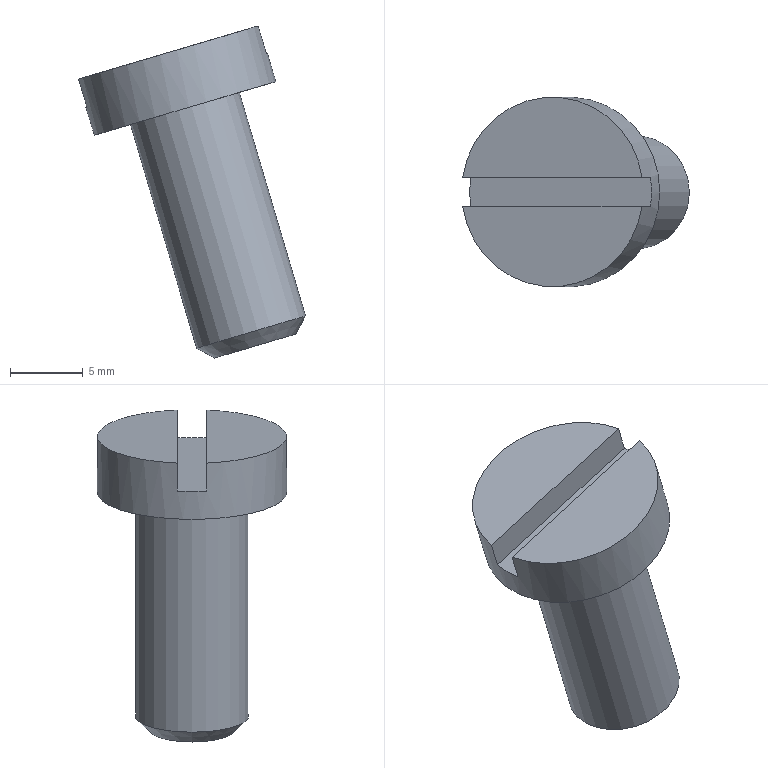Component | NX | SCREW_M8 | 1 solid | 10 faces | box 15.56 x 13 x 22.78 mm | volume 1277 mm3 | plane 7 | cylinder 2 | cone 1 | commonest cylinder face diameters 13 x1 7.785 x1
STEP:
#1=CARTESIAN_POINT('',(0.,0.,0.));
#2=DIRECTION('',(0.,0.,1.));
#3=DIRECTION('',(1.,0.,0.));
#4=AXIS2_PLACEMENT_3D('',#1,#2,#3);
#5=CARTESIAN_POINT('',(95.853,-1.,167.137));
#6=VERTEX_POINT('',#5);
#7=CARTESIAN_POINT('',(108.171,-1.,170.779));
#8=VERTEX_POINT('',#7);
#9=CARTESIAN_POINT('',(102.012,0.,168.958));
#10=DIRECTION('',(-0.2835,0.,0.959));
#11=DIRECTION('',(0.959,0.,0.2835));
#12=AXIS2_PLACEMENT_3D('',#9,#10,#11);
#13=CIRCLE('',#12,6.5);
#14=CARTESIAN_POINT('',(102.012,0.,168.958));
#15=DIRECTION('',(-0.2835,0.,0.959));
#16=DIRECTION('',(0.959,0.,0.2835));
#17=AXIS2_PLACEMENT_3D('',#14,#15,#16);
#18=PLANE('',#17);
#19=CARTESIAN_POINT('',(0.,0.));
#20=DIRECTION('',(1.,0.));
#21=AXIS2_PLACEMENT_2D('',#19,#20);
#22=CIRCLE('',#21,6.5);
#23=(GEOMETRIC_REPRESENTATION_CONTEXT(2)PARAMETRIC_REPRESENTATION_CONTEXT()REPRESENTATION_CONTEXT('',''));
#24=DEFINITIONAL_REPRESENTATION('',(#22),#23);
#25=PCURVE('',#18,#24);
#26=CARTESIAN_POINT('',(103.146,0.,165.122));
#27=DIRECTION('',(-0.2835,0.,0.959));
#28=DIRECTION('',(0.959,0.,0.2835));
#29=AXIS2_PLACEMENT_3D('',#26,#27,#28);
#30=CYLINDRICAL_SURFACE('',#29,6.5);
#31=CARTESIAN_POINT('',(0.,4.));
#32=DIRECTION('',(1.,0.));
#33=VECTOR('',#32,1.);
#34=LINE('',#31,#33);
#35=(GEOMETRIC_REPRESENTATION_CONTEXT(2)PARAMETRIC_REPRESENTATION_CONTEXT()REPRESENTATION_CONTEXT('',''));
#36=DEFINITIONAL_REPRESENTATION('',(#34),#35);
#37=PCURVE('',#30,#36);
#38=SURFACE_CURVE('',#13,(#25,#37),.PCURVE_S1.);
#39=EDGE_CURVE('',#6,#8,#38,.T.);
#40=ORIENTED_EDGE('',*,*,#39,.T.);
#41=CARTESIAN_POINT('',(111.193,-1.,171.672));
#42=DIRECTION('',(-0.959,0.,-0.2835));
#43=VECTOR('',#42,1.);
#44=LINE('',#41,#43);
#45=CARTESIAN_POINT('',(9.574,-1.));
#46=DIRECTION('',(-1.,0.));
#47=VECTOR('',#46,1.);
#48=LINE('',#45,#47);
#49=(GEOMETRIC_REPRESENTATION_CONTEXT(2)PARAMETRIC_REPRESENTATION_CONTEXT()REPRESENTATION_CONTEXT('',''));
#50=DEFINITIONAL_REPRESENTATION('',(#48),#49);
#51=PCURVE('',#18,#50);
#52=CARTESIAN_POINT('',(111.76,-1.,169.754));
#53=DIRECTION('',(0.,1.,0.));
#54=DIRECTION('',(-0.2835,0.,0.959));
#55=AXIS2_PLACEMENT_3D('',#52,#53,#54);
#56=PLANE('',#55);
#57=CARTESIAN_POINT('',(2.,0.));
#58=DIRECTION('',(0.,-1.));
#59=VECTOR('',#58,1.);
#60=LINE('',#57,#59);
#61=(GEOMETRIC_REPRESENTATION_CONTEXT(2)PARAMETRIC_REPRESENTATION_CONTEXT()REPRESENTATION_CONTEXT('',''));
#62=DEFINITIONAL_REPRESENTATION('',(#60),#61);
#63=PCURVE('',#56,#62);
#64=SURFACE_CURVE('',#44,(#51,#63),.PCURVE_S1.);
#65=EDGE_CURVE('',#8,#6,#64,.T.);
#66=ORIENTED_EDGE('',*,*,#65,.T.);
#67=EDGE_LOOP('',(#40,#66));
#68=FACE_BOUND('',#67,.T.);
#69=ADVANCED_FACE('',(#68),#18,.T.);
#70=CARTESIAN_POINT('',(108.171,1.,170.779));
#71=VERTEX_POINT('',#70);
#72=CARTESIAN_POINT('',(95.853,1.,167.137));
#73=VERTEX_POINT('',#72);
#74=CARTESIAN_POINT('',(102.012,0.,168.958));
#75=DIRECTION('',(-0.2835,0.,0.959));
#76=DIRECTION('',(0.959,0.,0.2835));
#77=AXIS2_PLACEMENT_3D('',#74,#75,#76);
#78=CIRCLE('',#77,6.5);
#79=CARTESIAN_POINT('',(102.012,0.,168.958));
#80=DIRECTION('',(-0.2835,0.,0.959));
#81=DIRECTION('',(0.959,0.,0.2835));
#82=AXIS2_PLACEMENT_3D('',#79,#80,#81);
#83=PLANE('',#82);
#84=CARTESIAN_POINT('',(0.,0.));
#85=DIRECTION('',(1.,0.));
#86=AXIS2_PLACEMENT_2D('',#84,#85);
#87=CIRCLE('',#86,6.5);
#88=(GEOMETRIC_REPRESENTATION_CONTEXT(2)PARAMETRIC_REPRESENTATION_CONTEXT()REPRESENTATION_CONTEXT('',''));
#89=DEFINITIONAL_REPRESENTATION('',(#87),#88);
#90=PCURVE('',#83,#89);
#91=CARTESIAN_POINT('',(-0.,4.));
#92=DIRECTION('',(1.,-0.));
#93=VECTOR('',#92,1.);
#94=LINE('',#91,#93);
#95=(GEOMETRIC_REPRESENTATION_CONTEXT(2)PARAMETRIC_REPRESENTATION_CONTEXT()REPRESENTATION_CONTEXT('',''));
#96=DEFINITIONAL_REPRESENTATION('',(#94),#95);
#97=PCURVE('',#30,#96);
#98=SURFACE_CURVE('',#78,(#90,#97),.PCURVE_S1.);
#99=EDGE_CURVE('',#71,#73,#98,.T.);
#100=ORIENTED_EDGE('',*,*,#99,.T.);
#101=CARTESIAN_POINT('',(92.831,1.,166.243));
#102=DIRECTION('',(0.959,0.,0.2835));
#103=VECTOR('',#102,1.);
#104=LINE('',#101,#103);
#105=CARTESIAN_POINT('',(-9.574,1.));
#106=DIRECTION('',(1.,0.));
#107=VECTOR('',#106,1.);
#108=LINE('',#105,#107);
#109=(GEOMETRIC_REPRESENTATION_CONTEXT(2)PARAMETRIC_REPRESENTATION_CONTEXT()REPRESENTATION_CONTEXT('',''));
#110=DEFINITIONAL_REPRESENTATION('',(#108),#109);
#111=PCURVE('',#83,#110);
#112=CARTESIAN_POINT('',(93.398,1.,164.325));
#113=DIRECTION('',(0.,-1.,0.));
#114=DIRECTION('',(0.2835,0.,-0.959));
#115=AXIS2_PLACEMENT_3D('',#112,#113,#114);
#116=PLANE('',#115);
#117=CARTESIAN_POINT('',(-2.,-0.));
#118=DIRECTION('',(0.,1.));
#119=VECTOR('',#118,1.);
#120=LINE('',#117,#119);
#121=(GEOMETRIC_REPRESENTATION_CONTEXT(2)PARAMETRIC_REPRESENTATION_CONTEXT()REPRESENTATION_CONTEXT('',''));
#122=DEFINITIONAL_REPRESENTATION('',(#120),#121);
#123=PCURVE('',#116,#122);
#124=SURFACE_CURVE('',#104,(#111,#123),.PCURVE_S1.);
#125=EDGE_CURVE('',#73,#71,#124,.T.);
#126=ORIENTED_EDGE('',*,*,#125,.T.);
#127=EDGE_LOOP('',(#100,#126));
#128=FACE_BOUND('',#127,.T.);
#129=ADVANCED_FACE('',(#128),#83,.T.);
#130=CARTESIAN_POINT('',(109.38,0.,166.965));
#131=VERTEX_POINT('',#130);
#132=CARTESIAN_POINT('',(103.146,0.,165.122));
#133=DIRECTION('',(-0.2835,0.,0.959));
#134=DIRECTION('',(0.959,0.,0.2835));
#135=AXIS2_PLACEMENT_3D('',#132,#133,#134);
#136=CIRCLE('',#135,6.5);
#137=CARTESIAN_POINT('',(0.,0.));
#138=DIRECTION('',(1.,0.));
#139=VECTOR('',#138,1.);
#140=LINE('',#137,#139);
#141=(GEOMETRIC_REPRESENTATION_CONTEXT(2)PARAMETRIC_REPRESENTATION_CONTEXT()REPRESENTATION_CONTEXT('',''));
#142=DEFINITIONAL_REPRESENTATION('',(#140),#141);
#143=PCURVE('',#30,#142);
#144=CARTESIAN_POINT('',(103.146,0.,165.122));
#145=DIRECTION('',(0.2835,0.,-0.959));
#146=DIRECTION('',(-0.959,0.,-0.2835));
#147=AXIS2_PLACEMENT_3D('',#144,#145,#146);
#148=PLANE('',#147);
#149=CARTESIAN_POINT('',(-6.5,0.));
#150=CARTESIAN_POINT('',(-6.5,11.258));
#151=CARTESIAN_POINT('',(3.25,5.629));
#152=CARTESIAN_POINT('',(13.,0.));
#153=CARTESIAN_POINT('',(3.25,-5.629));
#154=CARTESIAN_POINT('',(-6.5,-11.258));
#155=CARTESIAN_POINT('',(-6.5,0.));
#156=(BOUNDED_CURVE()B_SPLINE_CURVE(2,(#149,#150,#151,#152,#153,#154,#155),.UNSPECIFIED.,.T.,.F.)B_SPLINE_CURVE_WITH_KNOTS((1,2,2,2,2,1),(-2.094,0.,2.094,4.189,6.283,8.378),.UNSPECIFIED.)CURVE()GEOMETRIC_REPRESENTATION_ITEM()RATIONAL_B_SPLINE_CURVE((1.,0.5,1.,0.5,1.,0.5,1.))REPRESENTATION_ITEM(''));
#157=(GEOMETRIC_REPRESENTATION_CONTEXT(2)PARAMETRIC_REPRESENTATION_CONTEXT()REPRESENTATION_CONTEXT('',''));
#158=DEFINITIONAL_REPRESENTATION('',(#156),#157);
#159=PCURVE('',#148,#158);
#160=SURFACE_CURVE('',#136,(#143,#159),.PCURVE_S1.);
#161=EDGE_CURVE('',#131,#131,#160,.T.);
#162=ORIENTED_EDGE('',*,*,#161,.T.);
#163=CARTESIAN_POINT('',(108.812,0.,168.883));
#164=VERTEX_POINT('',#163);
#165=CARTESIAN_POINT('',(109.38,0.,166.965));
#166=CARTESIAN_POINT('',(108.812,0.,168.883));
#167=B_SPLINE_CURVE_WITH_KNOTS('',1,(#165,#166),.UNSPECIFIED.,.F.,.F.,(2,2),(0.,2.),.PIECEWISE_BEZIER_KNOTS.);
#168=CARTESIAN_POINT('',(6.283,0.));
#169=DIRECTION('',(0.,1.));
#170=VECTOR('',#169,1.);
#171=LINE('',#168,#170);
#172=(GEOMETRIC_REPRESENTATION_CONTEXT(2)PARAMETRIC_REPRESENTATION_CONTEXT()REPRESENTATION_CONTEXT('',''));
#173=DEFINITIONAL_REPRESENTATION('',(#171),#172);
#174=PCURVE('',#30,#173);
#175=CARTESIAN_POINT('',(0.,0.));
#176=DIRECTION('',(0.,1.));
#177=VECTOR('',#176,1.);
#178=LINE('',#175,#177);
#179=(GEOMETRIC_REPRESENTATION_CONTEXT(2)PARAMETRIC_REPRESENTATION_CONTEXT()REPRESENTATION_CONTEXT('',''));
#180=DEFINITIONAL_REPRESENTATION('',(#178),#179);
#181=PCURVE('',#30,#180);
#182=SEAM_CURVE('',#167,(#174,#181),.PCURVE_S1.);
#183=EDGE_CURVE('',#131,#164,#182,.T.);
#184=ORIENTED_EDGE('',*,*,#183,.T.);
#185=CARTESIAN_POINT('',(108.738,-1.,168.861));
#186=VERTEX_POINT('',#185);
#187=CARTESIAN_POINT('',(102.579,0.,167.04));
#188=DIRECTION('',(-0.2835,0.,0.959));
#189=DIRECTION('',(-0.959,0.,-0.2835));
#190=AXIS2_PLACEMENT_3D('',#187,#188,#189);
#191=CIRCLE('',#190,6.5);
#192=CARTESIAN_POINT('',(3.142,2.));
#193=DIRECTION('',(1.,0.));
#194=VECTOR('',#193,1.);
#195=LINE('',#192,#194);
#196=(GEOMETRIC_REPRESENTATION_CONTEXT(2)PARAMETRIC_REPRESENTATION_CONTEXT()REPRESENTATION_CONTEXT('',''));
#197=DEFINITIONAL_REPRESENTATION('',(#195),#196);
#198=PCURVE('',#30,#197);
#199=CARTESIAN_POINT('',(102.579,0.,167.04));
#200=DIRECTION('',(0.2835,0.,-0.959));
#201=DIRECTION('',(-0.959,0.,-0.2835));
#202=AXIS2_PLACEMENT_3D('',#199,#200,#201);
#203=PLANE('',#202);
#204=CARTESIAN_POINT('',(6.5,0.));
#205=CARTESIAN_POINT('',(6.5,-11.258));
#206=CARTESIAN_POINT('',(-3.25,-5.629));
#207=CARTESIAN_POINT('',(-13.,-0.));
#208=CARTESIAN_POINT('',(-3.25,5.629));
#209=CARTESIAN_POINT('',(6.5,11.258));
#210=CARTESIAN_POINT('',(6.5,0.));
#211=(BOUNDED_CURVE()B_SPLINE_CURVE(2,(#204,#205,#206,#207,#208,#209,#210),.UNSPECIFIED.,.T.,.F.)B_SPLINE_CURVE_WITH_KNOTS((1,2,2,2,2,1),(-2.094,0.,2.094,4.189,6.283,8.378),.UNSPECIFIED.)CURVE()GEOMETRIC_REPRESENTATION_ITEM()RATIONAL_B_SPLINE_CURVE((1.,0.5,1.,0.5,1.,0.5,1.))REPRESENTATION_ITEM(''));
#212=(GEOMETRIC_REPRESENTATION_CONTEXT(2)PARAMETRIC_REPRESENTATION_CONTEXT()REPRESENTATION_CONTEXT('',''));
#213=DEFINITIONAL_REPRESENTATION('',(#211),#212);
#214=PCURVE('',#203,#213);
#215=SURFACE_CURVE('',#191,(#198,#214),.PCURVE_S1.);
#216=EDGE_CURVE('',#186,#164,#215,.T.);
#217=ORIENTED_EDGE('',*,*,#216,.F.);
#218=CARTESIAN_POINT('',(109.305,-1.,166.943));
#219=DIRECTION('',(-0.2835,0.,0.959));
#220=VECTOR('',#219,1.);
#221=LINE('',#218,#220);
#222=CARTESIAN_POINT('',(6.129,-0.));
#223=DIRECTION('',(0.,1.));
#224=VECTOR('',#223,1.);
#225=LINE('',#222,#224);
#226=(GEOMETRIC_REPRESENTATION_CONTEXT(2)PARAMETRIC_REPRESENTATION_CONTEXT()REPRESENTATION_CONTEXT('',''));
#227=DEFINITIONAL_REPRESENTATION('',(#225),#226);
#228=PCURVE('',#30,#227);
#229=CARTESIAN_POINT('',(-2.,-3.151));
#230=DIRECTION('',(1.,0.));
#231=VECTOR('',#230,1.);
#232=LINE('',#229,#231);
#233=(GEOMETRIC_REPRESENTATION_CONTEXT(2)PARAMETRIC_REPRESENTATION_CONTEXT()REPRESENTATION_CONTEXT('',''));
#234=DEFINITIONAL_REPRESENTATION('',(#232),#233);
#235=PCURVE('',#56,#234);
#236=SURFACE_CURVE('',#221,(#228,#235),.PCURVE_S1.);
#237=EDGE_CURVE('',#186,#8,#236,.T.);
#238=ORIENTED_EDGE('',*,*,#237,.T.);
#239=ORIENTED_EDGE('',*,*,#39,.F.);
#240=CARTESIAN_POINT('',(96.42,-1.,165.219));
#241=VERTEX_POINT('',#240);
#242=CARTESIAN_POINT('',(96.987,-1.,163.301));
#243=DIRECTION('',(0.2835,0.,-0.959));
#244=VECTOR('',#243,1.);
#245=LINE('',#242,#244);
#246=CARTESIAN_POINT('',(3.296,-0.));
#247=DIRECTION('',(0.,-1.));
#248=VECTOR('',#247,1.);
#249=LINE('',#246,#248);
#250=(GEOMETRIC_REPRESENTATION_CONTEXT(2)PARAMETRIC_REPRESENTATION_CONTEXT()REPRESENTATION_CONTEXT('',''));
#251=DEFINITIONAL_REPRESENTATION('',(#249),#250);
#252=PCURVE('',#30,#251);
#253=CARTESIAN_POINT('',(-2.,-15.996));
#254=DIRECTION('',(-1.,0.));
#255=VECTOR('',#254,1.);
#256=LINE('',#253,#255);
#257=(GEOMETRIC_REPRESENTATION_CONTEXT(2)PARAMETRIC_REPRESENTATION_CONTEXT()REPRESENTATION_CONTEXT('',''));
#258=DEFINITIONAL_REPRESENTATION('',(#256),#257);
#259=PCURVE('',#56,#258);
#260=SURFACE_CURVE('',#245,(#252,#259),.PCURVE_S1.);
#261=EDGE_CURVE('',#6,#241,#260,.T.);
#262=ORIENTED_EDGE('',*,*,#261,.T.);
#263=CARTESIAN_POINT('',(96.42,1.,165.219));
#264=VERTEX_POINT('',#263);
#265=CARTESIAN_POINT('',(102.579,0.,167.04));
#266=DIRECTION('',(-0.2835,0.,0.959));
#267=DIRECTION('',(-0.959,0.,-0.2835));
#268=AXIS2_PLACEMENT_3D('',#265,#266,#267);
#269=CIRCLE('',#268,6.5);
#270=CARTESIAN_POINT('',(-3.142,2.));
#271=DIRECTION('',(1.,0.));
#272=VECTOR('',#271,1.);
#273=LINE('',#270,#272);
#274=(GEOMETRIC_REPRESENTATION_CONTEXT(2)PARAMETRIC_REPRESENTATION_CONTEXT()REPRESENTATION_CONTEXT('',''));
#275=DEFINITIONAL_REPRESENTATION('',(#273),#274);
#276=PCURVE('',#30,#275);
#277=CARTESIAN_POINT('',(6.5,0.));
#278=CARTESIAN_POINT('',(6.5,-11.258));
#279=CARTESIAN_POINT('',(-3.25,-5.629));
#280=CARTESIAN_POINT('',(-13.,-0.));
#281=CARTESIAN_POINT('',(-3.25,5.629));
#282=CARTESIAN_POINT('',(6.5,11.258));
#283=CARTESIAN_POINT('',(6.5,0.));
#284=(BOUNDED_CURVE()B_SPLINE_CURVE(2,(#277,#278,#279,#280,#281,#282,#283),.UNSPECIFIED.,.T.,.F.)B_SPLINE_CURVE_WITH_KNOTS((1,2,2,2,2,1),(-2.094,0.,2.094,4.189,6.283,8.378),.UNSPECIFIED.)CURVE()GEOMETRIC_REPRESENTATION_ITEM()RATIONAL_B_SPLINE_CURVE((1.,0.5,1.,0.5,1.,0.5,1.))REPRESENTATION_ITEM(''));
#285=(GEOMETRIC_REPRESENTATION_CONTEXT(2)PARAMETRIC_REPRESENTATION_CONTEXT()REPRESENTATION_CONTEXT('',''));
#286=DEFINITIONAL_REPRESENTATION('',(#284),#285);
#287=PCURVE('',#203,#286);
#288=SURFACE_CURVE('',#269,(#276,#287),.PCURVE_S1.);
#289=EDGE_CURVE('',#264,#241,#288,.T.);
#290=ORIENTED_EDGE('',*,*,#289,.F.);
#291=CARTESIAN_POINT('',(96.987,1.,163.301));
#292=DIRECTION('',(-0.2835,0.,0.959));
#293=VECTOR('',#292,1.);
#294=LINE('',#291,#293);
#295=CARTESIAN_POINT('',(2.987,-0.));
#296=DIRECTION('',(0.,1.));
#297=VECTOR('',#296,1.);
#298=LINE('',#295,#297);
#299=(GEOMETRIC_REPRESENTATION_CONTEXT(2)PARAMETRIC_REPRESENTATION_CONTEXT()REPRESENTATION_CONTEXT('',''));
#300=DEFINITIONAL_REPRESENTATION('',(#298),#299);
#301=PCURVE('',#30,#300);
#302=CARTESIAN_POINT('',(2.,3.151));
#303=DIRECTION('',(-1.,0.));
#304=VECTOR('',#303,1.);
#305=LINE('',#302,#304);
#306=(GEOMETRIC_REPRESENTATION_CONTEXT(2)PARAMETRIC_REPRESENTATION_CONTEXT()REPRESENTATION_CONTEXT('',''));
#307=DEFINITIONAL_REPRESENTATION('',(#305),#306);
#308=PCURVE('',#116,#307);
#309=SURFACE_CURVE('',#294,(#301,#308),.PCURVE_S1.);
#310=EDGE_CURVE('',#264,#73,#309,.T.);
#311=ORIENTED_EDGE('',*,*,#310,.T.);
#312=ORIENTED_EDGE('',*,*,#99,.F.);
#313=CARTESIAN_POINT('',(108.738,1.,168.861));
#314=VERTEX_POINT('',#313);
#315=CARTESIAN_POINT('',(109.305,1.,166.943));
#316=DIRECTION('',(0.2835,0.,-0.959));
#317=VECTOR('',#316,1.);
#318=LINE('',#315,#317);
#319=CARTESIAN_POINT('',(0.1545,-0.));
#320=DIRECTION('',(0.,-1.));
#321=VECTOR('',#320,1.);
#322=LINE('',#319,#321);
#323=(GEOMETRIC_REPRESENTATION_CONTEXT(2)PARAMETRIC_REPRESENTATION_CONTEXT()REPRESENTATION_CONTEXT('',''));
#324=DEFINITIONAL_REPRESENTATION('',(#322),#323);
#325=PCURVE('',#30,#324);
#326=CARTESIAN_POINT('',(2.,15.996));
#327=DIRECTION('',(1.,0.));
#328=VECTOR('',#327,1.);
#329=LINE('',#326,#328);
#330=(GEOMETRIC_REPRESENTATION_CONTEXT(2)PARAMETRIC_REPRESENTATION_CONTEXT()REPRESENTATION_CONTEXT('',''));
#331=DEFINITIONAL_REPRESENTATION('',(#329),#330);
#332=PCURVE('',#116,#331);
#333=SURFACE_CURVE('',#318,(#325,#332),.PCURVE_S1.);
#334=EDGE_CURVE('',#71,#314,#333,.T.);
#335=ORIENTED_EDGE('',*,*,#334,.T.);
#336=CARTESIAN_POINT('',(102.579,0.,167.04));
#337=DIRECTION('',(-0.2835,0.,0.959));
#338=DIRECTION('',(-0.959,0.,-0.2835));
#339=AXIS2_PLACEMENT_3D('',#336,#337,#338);
#340=CIRCLE('',#339,6.5);
#341=CARTESIAN_POINT('',(-3.142,2.));
#342=DIRECTION('',(1.,0.));
#343=VECTOR('',#342,1.);
#344=LINE('',#341,#343);
#345=(GEOMETRIC_REPRESENTATION_CONTEXT(2)PARAMETRIC_REPRESENTATION_CONTEXT()REPRESENTATION_CONTEXT('',''));
#346=DEFINITIONAL_REPRESENTATION('',(#344),#345);
#347=PCURVE('',#30,#346);
#348=CARTESIAN_POINT('',(6.5,0.));
#349=CARTESIAN_POINT('',(6.5,-11.258));
#350=CARTESIAN_POINT('',(-3.25,-5.629));
#351=CARTESIAN_POINT('',(-13.,-0.));
#352=CARTESIAN_POINT('',(-3.25,5.629));
#353=CARTESIAN_POINT('',(6.5,11.258));
#354=CARTESIAN_POINT('',(6.5,0.));
#355=(BOUNDED_CURVE()B_SPLINE_CURVE(2,(#348,#349,#350,#351,#352,#353,#354),.UNSPECIFIED.,.T.,.F.)B_SPLINE_CURVE_WITH_KNOTS((1,2,2,2,2,1),(-2.094,0.,2.094,4.189,6.283,8.378),.UNSPECIFIED.)CURVE()GEOMETRIC_REPRESENTATION_ITEM()RATIONAL_B_SPLINE_CURVE((1.,0.5,1.,0.5,1.,0.5,1.))REPRESENTATION_ITEM(''));
#356=(GEOMETRIC_REPRESENTATION_CONTEXT(2)PARAMETRIC_REPRESENTATION_CONTEXT()REPRESENTATION_CONTEXT('',''));
#357=DEFINITIONAL_REPRESENTATION('',(#355),#356);
#358=PCURVE('',#203,#357);
#359=SURFACE_CURVE('',#340,(#347,#358),.PCURVE_S1.);
#360=EDGE_CURVE('',#164,#314,#359,.T.);
#361=ORIENTED_EDGE('',*,*,#360,.F.);
#362=ORIENTED_EDGE('',*,*,#183,.F.);
#363=EDGE_LOOP('',(#162,#184,#217,#238,#239,#262,#290,#311,#312,#335,#361,#362));
#364=FACE_BOUND('',#363,.T.);
#365=ADVANCED_FACE('',(#364),#30,.T.);
#366=CARTESIAN_POINT('',(105.193,0.,147.999));
#367=VERTEX_POINT('',#366);
#368=CARTESIAN_POINT('',(107.967,0.,148.82));
#369=DIRECTION('',(0.2835,0.,-0.959));
#370=DIRECTION('',(-0.959,0.,-0.2835));
#371=AXIS2_PLACEMENT_3D('',#368,#369,#370);
#372=CIRCLE('',#371,2.893);
#373=CARTESIAN_POINT('',(107.967,0.,148.82));
#374=DIRECTION('',(0.2835,0.,-0.959));
#375=DIRECTION('',(-0.959,0.,-0.2835));
#376=AXIS2_PLACEMENT_3D('',#373,#374,#375);
#377=PLANE('',#376);
#378=CARTESIAN_POINT('',(0.,0.));
#379=DIRECTION('',(1.,0.));
#380=AXIS2_PLACEMENT_2D('',#378,#379);
#381=CIRCLE('',#380,2.893);
#382=(GEOMETRIC_REPRESENTATION_CONTEXT(2)PARAMETRIC_REPRESENTATION_CONTEXT()REPRESENTATION_CONTEXT('',''));
#383=DEFINITIONAL_REPRESENTATION('',(#381),#382);
#384=PCURVE('',#377,#383);
#385=CARTESIAN_POINT('',(107.683,0.,149.779));
#386=DIRECTION('',(-0.2835,0.,0.959));
#387=DIRECTION('',(0.959,0.,0.2835));
#388=AXIS2_PLACEMENT_3D('',#385,#386,#387);
#389=CONICAL_SURFACE('',#388,3.893,0.7854);
#390=CARTESIAN_POINT('',(9.425,-1.));
#391=DIRECTION('',(-1.,0.));
#392=VECTOR('',#391,1.);
#393=LINE('',#390,#392);
#394=(GEOMETRIC_REPRESENTATION_CONTEXT(2)PARAMETRIC_REPRESENTATION_CONTEXT()REPRESENTATION_CONTEXT('',''));
#395=DEFINITIONAL_REPRESENTATION('',(#393),#394);
#396=PCURVE('',#389,#395);
#397=SURFACE_CURVE('',#372,(#384,#396),.PCURVE_S1.);
#398=EDGE_CURVE('',#367,#367,#397,.T.);
#399=ORIENTED_EDGE('',*,*,#398,.T.);
#400=EDGE_LOOP('',(#399));
#401=FACE_BOUND('',#400,.T.);
#402=ADVANCED_FACE('',(#401),#377,.T.);
#403=CARTESIAN_POINT('',(103.95,0.,148.675));
#404=VERTEX_POINT('',#403);
#405=CARTESIAN_POINT('',(111.416,0.,150.882));
#406=VERTEX_POINT('',#405);
#407=CARTESIAN_POINT('',(107.683,0.,149.779));
#408=DIRECTION('',(-0.2835,0.,0.959));
#409=DIRECTION('',(-0.959,0.,-0.2835));
#410=AXIS2_PLACEMENT_3D('',#407,#408,#409);
#411=CIRCLE('',#410,3.893);
#412=CARTESIAN_POINT('',(107.967,0.,148.82));
#413=DIRECTION('',(-0.2835,0.,0.959));
#414=DIRECTION('',(0.959,0.,0.2835));
#415=AXIS2_PLACEMENT_3D('',#412,#413,#414);
#416=CYLINDRICAL_SURFACE('',#415,3.893);
#417=CARTESIAN_POINT('',(3.142,1.));
#418=DIRECTION('',(1.,0.));
#419=VECTOR('',#418,1.);
#420=LINE('',#417,#419);
#421=(GEOMETRIC_REPRESENTATION_CONTEXT(2)PARAMETRIC_REPRESENTATION_CONTEXT()REPRESENTATION_CONTEXT('',''));
#422=DEFINITIONAL_REPRESENTATION('',(#420),#421);
#423=PCURVE('',#416,#422);
#424=CARTESIAN_POINT('',(3.142,-0.));
#425=DIRECTION('',(1.,0.));
#426=VECTOR('',#425,1.);
#427=LINE('',#424,#426);
#428=(GEOMETRIC_REPRESENTATION_CONTEXT(2)PARAMETRIC_REPRESENTATION_CONTEXT()REPRESENTATION_CONTEXT('',''));
#429=DEFINITIONAL_REPRESENTATION('',(#427),#428);
#430=PCURVE('',#389,#429);
#431=SURFACE_CURVE('',#411,(#423,#430),.PCURVE_S1.);
#432=EDGE_CURVE('',#404,#406,#431,.T.);
#433=ORIENTED_EDGE('',*,*,#432,.T.);
#434=CARTESIAN_POINT('',(106.879,0.,166.226));
#435=VERTEX_POINT('',#434);
#436=CARTESIAN_POINT('',(111.416,0.,150.882));
#437=CARTESIAN_POINT('',(106.879,0.,166.226));
#438=B_SPLINE_CURVE_WITH_KNOTS('',1,(#436,#437),.UNSPECIFIED.,.F.,.F.,(2,2),(1.,17.),.PIECEWISE_BEZIER_KNOTS.);
#439=CARTESIAN_POINT('',(6.283,0.));
#440=DIRECTION('',(0.,1.));
#441=VECTOR('',#440,1.);
#442=LINE('',#439,#441);
#443=(GEOMETRIC_REPRESENTATION_CONTEXT(2)PARAMETRIC_REPRESENTATION_CONTEXT()REPRESENTATION_CONTEXT('',''));
#444=DEFINITIONAL_REPRESENTATION('',(#442),#443);
#445=PCURVE('',#416,#444);
#446=CARTESIAN_POINT('',(0.,0.));
#447=DIRECTION('',(0.,1.));
#448=VECTOR('',#447,1.);
#449=LINE('',#446,#448);
#450=(GEOMETRIC_REPRESENTATION_CONTEXT(2)PARAMETRIC_REPRESENTATION_CONTEXT()REPRESENTATION_CONTEXT('',''));
#451=DEFINITIONAL_REPRESENTATION('',(#449),#450);
#452=PCURVE('',#416,#451);
#453=SEAM_CURVE('',#438,(#445,#452),.PCURVE_S1.);
#454=EDGE_CURVE('',#406,#435,#453,.T.);
#455=ORIENTED_EDGE('',*,*,#454,.T.);
#456=CARTESIAN_POINT('',(103.146,0.,165.122));
#457=DIRECTION('',(0.2835,0.,-0.959));
#458=DIRECTION('',(0.959,0.,0.2835));
#459=AXIS2_PLACEMENT_3D('',#456,#457,#458);
#460=CIRCLE('',#459,3.893);
#461=CARTESIAN_POINT('',(6.283,17.));
#462=DIRECTION('',(-1.,0.));
#463=VECTOR('',#462,1.);
#464=LINE('',#461,#463);
#465=(GEOMETRIC_REPRESENTATION_CONTEXT(2)PARAMETRIC_REPRESENTATION_CONTEXT()REPRESENTATION_CONTEXT('',''));
#466=DEFINITIONAL_REPRESENTATION('',(#464),#465);
#467=PCURVE('',#416,#466);
#468=CARTESIAN_POINT('',(0.,0.));
#469=DIRECTION('',(-1.,0.));
#470=AXIS2_PLACEMENT_2D('',#468,#469);
#471=CIRCLE('',#470,3.893);
#472=(GEOMETRIC_REPRESENTATION_CONTEXT(2)PARAMETRIC_REPRESENTATION_CONTEXT()REPRESENTATION_CONTEXT('',''));
#473=DEFINITIONAL_REPRESENTATION('',(#471),#472);
#474=PCURVE('',#148,#473);
#475=SURFACE_CURVE('',#460,(#467,#474),.PCURVE_S1.);
#476=EDGE_CURVE('',#435,#435,#475,.T.);
#477=ORIENTED_EDGE('',*,*,#476,.T.);
#478=ORIENTED_EDGE('',*,*,#454,.F.);
#479=CARTESIAN_POINT('',(107.683,0.,149.779));
#480=DIRECTION('',(-0.2835,0.,0.959));
#481=DIRECTION('',(-0.959,0.,-0.2835));
#482=AXIS2_PLACEMENT_3D('',#479,#480,#481);
#483=CIRCLE('',#482,3.893);
#484=CARTESIAN_POINT('',(-3.142,1.));
#485=DIRECTION('',(1.,0.));
#486=VECTOR('',#485,1.);
#487=LINE('',#484,#486);
#488=(GEOMETRIC_REPRESENTATION_CONTEXT(2)PARAMETRIC_REPRESENTATION_CONTEXT()REPRESENTATION_CONTEXT('',''));
#489=DEFINITIONAL_REPRESENTATION('',(#487),#488);
#490=PCURVE('',#416,#489);
#491=CARTESIAN_POINT('',(3.142,-0.));
#492=DIRECTION('',(1.,0.));
#493=VECTOR('',#492,1.);
#494=LINE('',#491,#493);
#495=(GEOMETRIC_REPRESENTATION_CONTEXT(2)PARAMETRIC_REPRESENTATION_CONTEXT()REPRESENTATION_CONTEXT('',''));
#496=DEFINITIONAL_REPRESENTATION('',(#494),#495);
#497=PCURVE('',#389,#496);
#498=SURFACE_CURVE('',#483,(#490,#497),.PCURVE_S1.);
#499=EDGE_CURVE('',#406,#404,#498,.T.);
#500=ORIENTED_EDGE('',*,*,#499,.T.);
#501=EDGE_LOOP('',(#433,#455,#477,#478,#500));
#502=FACE_BOUND('',#501,.T.);
#503=ADVANCED_FACE('',(#502),#416,.T.);
#504=ORIENTED_EDGE('',*,*,#476,.F.);
#505=EDGE_LOOP('',(#504));
#506=FACE_BOUND('',#505,.T.);
#507=ORIENTED_EDGE('',*,*,#161,.F.);
#508=EDGE_LOOP('',(#507));
#509=FACE_BOUND('',#508,.T.);
#510=ADVANCED_FACE('',(#506,#509),#148,.T.);
#511=ORIENTED_EDGE('',*,*,#398,.F.);
#512=CARTESIAN_POINT('',(105.193,0.,147.999));
#513=CARTESIAN_POINT('',(103.95,0.,148.675));
#514=B_SPLINE_CURVE_WITH_KNOTS('',1,(#512,#513),.UNSPECIFIED.,.F.,.F.,(2,2),(-1.414,-0.),.PIECEWISE_BEZIER_KNOTS.);
#515=CARTESIAN_POINT('',(9.425,0.));
#516=DIRECTION('',(0.,1.));
#517=VECTOR('',#516,1.);
#518=LINE('',#515,#517);
#519=(GEOMETRIC_REPRESENTATION_CONTEXT(2)PARAMETRIC_REPRESENTATION_CONTEXT()REPRESENTATION_CONTEXT('',''));
#520=DEFINITIONAL_REPRESENTATION('',(#518),#519);
#521=PCURVE('',#389,#520);
#522=CARTESIAN_POINT('',(3.142,0.));
#523=DIRECTION('',(0.,1.));
#524=VECTOR('',#523,1.);
#525=LINE('',#522,#524);
#526=(GEOMETRIC_REPRESENTATION_CONTEXT(2)PARAMETRIC_REPRESENTATION_CONTEXT()REPRESENTATION_CONTEXT('',''));
#527=DEFINITIONAL_REPRESENTATION('',(#525),#526);
#528=PCURVE('',#389,#527);
#529=SEAM_CURVE('',#514,(#521,#528),.PCURVE_S1.);
#530=EDGE_CURVE('',#367,#404,#529,.T.);
#531=ORIENTED_EDGE('',*,*,#530,.T.);
#532=ORIENTED_EDGE('',*,*,#499,.F.);
#533=ORIENTED_EDGE('',*,*,#432,.F.);
#534=ORIENTED_EDGE('',*,*,#530,.F.);
#535=EDGE_LOOP('',(#511,#531,#532,#533,#534));
#536=FACE_BOUND('',#535,.T.);
#537=ADVANCED_FACE('',(#536),#389,.T.);
#538=ORIENTED_EDGE('',*,*,#65,.F.);
#539=ORIENTED_EDGE('',*,*,#237,.F.);
#540=CARTESIAN_POINT('',(111.76,-1.,169.754));
#541=DIRECTION('',(0.959,0.,0.2835));
#542=VECTOR('',#541,1.);
#543=LINE('',#540,#542);
#544=CARTESIAN_POINT('',(0.,0.));
#545=DIRECTION('',(0.,1.));
#546=VECTOR('',#545,1.);
#547=LINE('',#544,#546);
#548=(GEOMETRIC_REPRESENTATION_CONTEXT(2)PARAMETRIC_REPRESENTATION_CONTEXT()REPRESENTATION_CONTEXT('',''));
#549=DEFINITIONAL_REPRESENTATION('',(#547),#548);
#550=PCURVE('',#56,#549);
#551=CARTESIAN_POINT('',(-9.574,-1.));
#552=DIRECTION('',(-1.,0.));
#553=VECTOR('',#552,1.);
#554=LINE('',#551,#553);
#555=(GEOMETRIC_REPRESENTATION_CONTEXT(2)PARAMETRIC_REPRESENTATION_CONTEXT()REPRESENTATION_CONTEXT('',''));
#556=DEFINITIONAL_REPRESENTATION('',(#554),#555);
#557=PCURVE('',#203,#556);
#558=SURFACE_CURVE('',#543,(#550,#557),.PCURVE_S1.);
#559=EDGE_CURVE('',#241,#186,#558,.T.);
#560=ORIENTED_EDGE('',*,*,#559,.F.);
#561=ORIENTED_EDGE('',*,*,#261,.F.);
#562=EDGE_LOOP('',(#538,#539,#560,#561));
#563=FACE_BOUND('',#562,.T.);
#564=ADVANCED_FACE('',(#563),#56,.T.);
#565=ORIENTED_EDGE('',*,*,#125,.F.);
#566=ORIENTED_EDGE('',*,*,#310,.F.);
#567=CARTESIAN_POINT('',(93.398,1.,164.325));
#568=DIRECTION('',(-0.959,0.,-0.2835));
#569=VECTOR('',#568,1.);
#570=LINE('',#567,#569);
#571=CARTESIAN_POINT('',(0.,0.));
#572=DIRECTION('',(0.,-1.));
#573=VECTOR('',#572,1.);
#574=LINE('',#571,#573);
#575=(GEOMETRIC_REPRESENTATION_CONTEXT(2)PARAMETRIC_REPRESENTATION_CONTEXT()REPRESENTATION_CONTEXT('',''));
#576=DEFINITIONAL_REPRESENTATION('',(#574),#575);
#577=PCURVE('',#116,#576);
#578=CARTESIAN_POINT('',(9.574,1.));
#579=DIRECTION('',(1.,0.));
#580=VECTOR('',#579,1.);
#581=LINE('',#578,#580);
#582=(GEOMETRIC_REPRESENTATION_CONTEXT(2)PARAMETRIC_REPRESENTATION_CONTEXT()REPRESENTATION_CONTEXT('',''));
#583=DEFINITIONAL_REPRESENTATION('',(#581),#582);
#584=PCURVE('',#203,#583);
#585=SURFACE_CURVE('',#570,(#577,#584),.PCURVE_S1.);
#586=EDGE_CURVE('',#314,#264,#585,.T.);
#587=ORIENTED_EDGE('',*,*,#586,.F.);
#588=ORIENTED_EDGE('',*,*,#334,.F.);
#589=EDGE_LOOP('',(#565,#566,#587,#588));
#590=FACE_BOUND('',#589,.T.);
#591=ADVANCED_FACE('',(#590),#116,.T.);
#592=ORIENTED_EDGE('',*,*,#216,.T.);
#593=ORIENTED_EDGE('',*,*,#360,.T.);
#594=ORIENTED_EDGE('',*,*,#586,.T.);
#595=ORIENTED_EDGE('',*,*,#289,.T.);
#596=ORIENTED_EDGE('',*,*,#559,.T.);
#597=EDGE_LOOP('',(#592,#593,#594,#595,#596));
#598=FACE_BOUND('',#597,.T.);
#599=ADVANCED_FACE('',(#598),#203,.F.);
#600=CLOSED_SHELL('',(#69,#129,#365,#402,#503,#510,#537,#564,#591,#599));
#601=MANIFOLD_SOLID_BREP('',#600);
#602=(LENGTH_UNIT()NAMED_UNIT(*)SI_UNIT(.MILLI.,.METRE.));
#603=UNCERTAINTY_MEASURE_WITH_UNIT(LENGTH_MEASURE(0.000002),#602,'','');
#604=(NAMED_UNIT(*)PLANE_ANGLE_UNIT()SI_UNIT($,.RADIAN.));
#605=(NAMED_UNIT(*)SI_UNIT($,.STERADIAN.)SOLID_ANGLE_UNIT());
#606=(GEOMETRIC_REPRESENTATION_CONTEXT(3)GLOBAL_UNCERTAINTY_ASSIGNED_CONTEXT((#603))GLOBAL_UNIT_ASSIGNED_CONTEXT((#602,#604,#605))REPRESENTATION_CONTEXT('',''));
#607=ADVANCED_BREP_SHAPE_REPRESENTATION('',(#4,#601),#606);